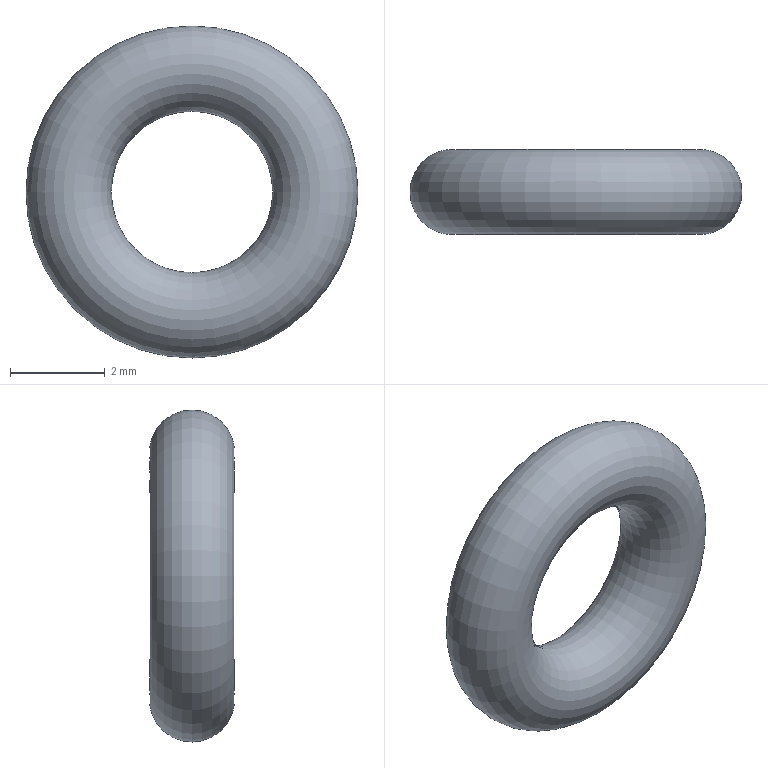Component | NX | O_RING_2 | 1 solid | 1 faces | box 7 x 1.8 x 7 mm | volume 42 mm3 | torus 1
STEP:
#1=CARTESIAN_POINT('',(0.,0.,0.));
#2=DIRECTION('',(0.,0.,1.));
#3=DIRECTION('',(1.,0.,0.));
#4=AXIS2_PLACEMENT_3D('',#1,#2,#3);
#5=CARTESIAN_POINT('',(13.994,-119.116,3.5));
#6=VERTEX_POINT('',#5);
#7=CARTESIAN_POINT('',(13.994,-119.116,2.6));
#8=DIRECTION('',(1.,0.,0.));
#9=DIRECTION('',(0.,0.,1.));
#10=AXIS2_PLACEMENT_3D('',#7,#8,#9);
#11=CIRCLE('',#10,0.9);
#12=CARTESIAN_POINT('',(13.994,-119.116,-0.));
#13=DIRECTION('',(0.,-1.,0.));
#14=DIRECTION('',(0.,0.,1.));
#15=AXIS2_PLACEMENT_3D('',#12,#13,#14);
#16=TOROIDAL_SURFACE('',#15,2.6,0.9);
#17=CARTESIAN_POINT('',(0.,0.));
#18=DIRECTION('',(0.,1.));
#19=VECTOR('',#18,1.);
#20=LINE('',#17,#19);
#21=(GEOMETRIC_REPRESENTATION_CONTEXT(2)PARAMETRIC_REPRESENTATION_CONTEXT()REPRESENTATION_CONTEXT('',''));
#22=DEFINITIONAL_REPRESENTATION('',(#20),#21);
#23=PCURVE('',#16,#22);
#24=CARTESIAN_POINT('',(6.283,0.));
#25=DIRECTION('',(0.,1.));
#26=VECTOR('',#25,1.);
#27=LINE('',#24,#26);
#28=(GEOMETRIC_REPRESENTATION_CONTEXT(2)PARAMETRIC_REPRESENTATION_CONTEXT()REPRESENTATION_CONTEXT('',''));
#29=DEFINITIONAL_REPRESENTATION('',(#27),#28);
#30=PCURVE('',#16,#29);
#31=SEAM_CURVE('',#11,(#23,#30),.PCURVE_S1.);
#32=EDGE_CURVE('',#6,#6,#31,.T.);
#33=ORIENTED_EDGE('',*,*,#32,.F.);
#34=CARTESIAN_POINT('',(13.994,-119.116,-0.));
#35=DIRECTION('',(0.,-1.,0.));
#36=DIRECTION('',(0.,0.,1.));
#37=AXIS2_PLACEMENT_3D('',#34,#35,#36);
#38=CIRCLE('',#37,3.5);
#39=CARTESIAN_POINT('',(0.,0.));
#40=DIRECTION('',(1.,0.));
#41=VECTOR('',#40,1.);
#42=LINE('',#39,#41);
#43=(GEOMETRIC_REPRESENTATION_CONTEXT(2)PARAMETRIC_REPRESENTATION_CONTEXT()REPRESENTATION_CONTEXT('',''));
#44=DEFINITIONAL_REPRESENTATION('',(#42),#43);
#45=PCURVE('',#16,#44);
#46=CARTESIAN_POINT('',(0.,6.283));
#47=DIRECTION('',(1.,0.));
#48=VECTOR('',#47,1.);
#49=LINE('',#46,#48);
#50=(GEOMETRIC_REPRESENTATION_CONTEXT(2)PARAMETRIC_REPRESENTATION_CONTEXT()REPRESENTATION_CONTEXT('',''));
#51=DEFINITIONAL_REPRESENTATION('',(#49),#50);
#52=PCURVE('',#16,#51);
#53=SEAM_CURVE('',#38,(#45,#52),.PCURVE_S1.);
#54=EDGE_CURVE('',#6,#6,#53,.T.);
#55=ORIENTED_EDGE('',*,*,#54,.T.);
#56=ORIENTED_EDGE('',*,*,#32,.T.);
#57=ORIENTED_EDGE('',*,*,#54,.F.);
#58=EDGE_LOOP('',(#33,#55,#56,#57));
#59=FACE_BOUND('',#58,.T.);
#60=ADVANCED_FACE('',(#59),#16,.T.);
#61=CLOSED_SHELL('',(#60));
#62=MANIFOLD_SOLID_BREP('',#61);
#63=(LENGTH_UNIT()NAMED_UNIT(*)SI_UNIT(.MILLI.,.METRE.));
#64=UNCERTAINTY_MEASURE_WITH_UNIT(LENGTH_MEASURE(0.0000001),#63,'','');
#65=(NAMED_UNIT(*)PLANE_ANGLE_UNIT()SI_UNIT($,.RADIAN.));
#66=(NAMED_UNIT(*)SI_UNIT($,.STERADIAN.)SOLID_ANGLE_UNIT());
#67=(GEOMETRIC_REPRESENTATION_CONTEXT(3)GLOBAL_UNCERTAINTY_ASSIGNED_CONTEXT((#64))GLOBAL_UNIT_ASSIGNED_CONTEXT((#63,#65,#66))REPRESENTATION_CONTEXT('',''));
#68=ADVANCED_BREP_SHAPE_REPRESENTATION('',(#4,#62),#67);